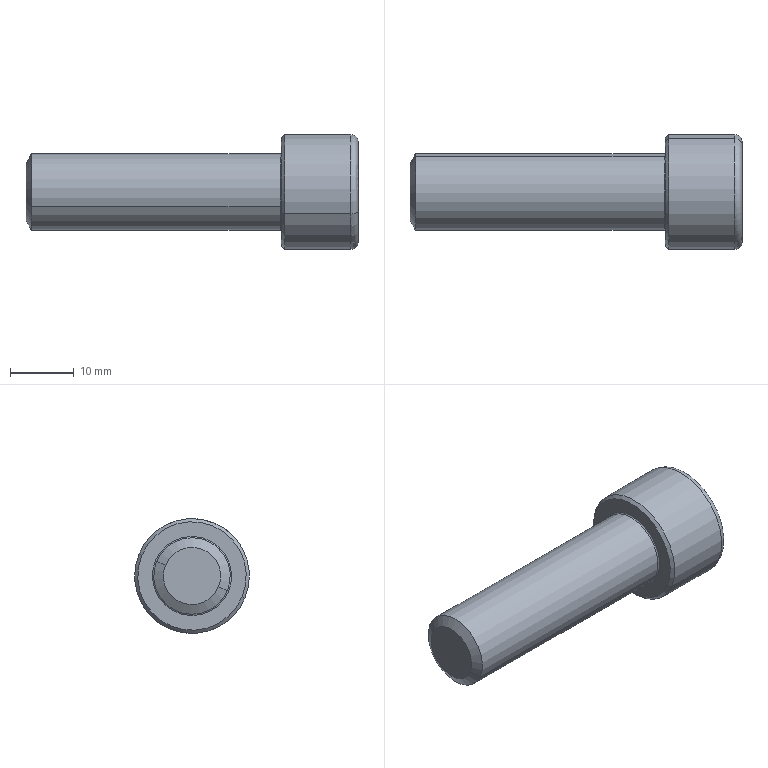Component | SolidWorks | M12_40_T70.1-1 | 1 solid | 28 faces | box 52 x 18 x 18 mm | volume 7021 mm3 | cone 10 | plane 10 | torus 4 | cylinder 4 | commonest cylinder face diameters 18 x2 12 x2 | material Plain Carbon Steel
STEP:
#1=COLOUR_RGB('',0.7922,0.8196,0.9333);
#2=FILL_AREA_STYLE_COLOUR('',#1);
#3=FILL_AREA_STYLE('',(#2));
#4=SURFACE_STYLE_FILL_AREA(#3);
#5=SURFACE_SIDE_STYLE('',(#4));
#6=SURFACE_STYLE_USAGE(.BOTH.,#5);
#7=PRESENTATION_STYLE_ASSIGNMENT((#6));
#8=CARTESIAN_POINT('',(0.122,0.3093,-1.967));
#9=VERTEX_POINT('',#8);
#10=CARTESIAN_POINT('',(0.122,-0.3093,-2.222));
#11=VERTEX_POINT('',#10);
#12=CARTESIAN_POINT('',(0.122,0.,-2.094));
#13=DIRECTION('',(-1.,0.,0.));
#14=DIRECTION('',(0.,-0.9242,-0.3818));
#15=AXIS2_PLACEMENT_3D('',#12,#13,#14);
#16=CIRCLE('',#15,0.3346);
#17=EDGE_CURVE('',#9,#11,#16,.T.);
#18=ORIENTED_EDGE('',*,*,#17,.F.);
#19=CARTESIAN_POINT('',(0.1417,0.3275,-1.959));
#20=VERTEX_POINT('',#19);
#21=CARTESIAN_POINT('',(0.1417,0.3275,-1.959));
#22=DIRECTION('',(0.7071,0.6535,0.27));
#23=VECTOR('',#22,39.37);
#24=LINE('',#21,#23);
#25=EDGE_CURVE('',#9,#20,#24,.T.);
#26=ORIENTED_EDGE('',*,*,#25,.T.);
#27=CARTESIAN_POINT('',(0.1417,-0.3275,-2.23));
#28=VERTEX_POINT('',#27);
#29=CARTESIAN_POINT('',(0.1417,0.,-2.094));
#30=DIRECTION('',(1.,0.,0.));
#31=DIRECTION('',(0.,-0.9242,-0.3818));
#32=AXIS2_PLACEMENT_3D('',#29,#30,#31);
#33=CIRCLE('',#32,0.3543);
#34=EDGE_CURVE('',#28,#20,#33,.T.);
#35=ORIENTED_EDGE('',*,*,#34,.F.);
#36=CARTESIAN_POINT('',(0.1417,-0.3275,-2.23));
#37=DIRECTION('',(0.7071,-0.6535,-0.27));
#38=VECTOR('',#37,39.37);
#39=LINE('',#36,#38);
#40=EDGE_CURVE('',#11,#28,#39,.T.);
#41=ORIENTED_EDGE('',*,*,#40,.F.);
#42=EDGE_LOOP('',(#18,#26,#35,#41));
#43=FACE_OUTER_BOUND('',#42,.T.);
#44=CARTESIAN_POINT('',(0.1417,0.,-2.094));
#45=DIRECTION('',(1.,0.,0.));
#46=DIRECTION('',(0.,-0.9242,-0.3818));
#47=AXIS2_PLACEMENT_3D('',#44,#45,#46);
#48=CONICAL_SURFACE('',#47,0.3543,0.7854);
#49=ADVANCED_FACE('',(#43),#48,.T.);
#50=CARTESIAN_POINT('',(0.5945,-0.2875,-2.213));
#51=VERTEX_POINT('',#50);
#52=CARTESIAN_POINT('',(0.5945,0.2875,-1.976));
#53=VERTEX_POINT('',#52);
#54=CARTESIAN_POINT('',(0.5945,0.,-2.094));
#55=DIRECTION('',(1.,0.,0.));
#56=DIRECTION('',(0.,0.9242,0.3818));
#57=AXIS2_PLACEMENT_3D('',#54,#55,#56);
#58=CIRCLE('',#57,0.311);
#59=EDGE_CURVE('',#51,#53,#58,.T.);
#60=ORIENTED_EDGE('',*,*,#59,.F.);
#61=CARTESIAN_POINT('',(0.5512,-0.3275,-2.23));
#62=VERTEX_POINT('',#61);
#63=CARTESIAN_POINT('',(0.5512,-0.2875,-2.213));
#64=DIRECTION('',(0.,0.3818,-0.9242));
#65=DIRECTION('',(0.,0.9242,0.3818));
#66=AXIS2_PLACEMENT_3D('',#63,#64,#65);
#67=CIRCLE('',#66,0.04331);
#68=EDGE_CURVE('',#51,#62,#67,.T.);
#69=ORIENTED_EDGE('',*,*,#68,.T.);
#70=CARTESIAN_POINT('',(0.5512,0.3275,-1.959));
#71=VERTEX_POINT('',#70);
#72=CARTESIAN_POINT('',(0.5512,0.,-2.094));
#73=DIRECTION('',(-1.,0.,0.));
#74=DIRECTION('',(0.,0.9242,0.3818));
#75=AXIS2_PLACEMENT_3D('',#72,#73,#74);
#76=CIRCLE('',#75,0.3543);
#77=EDGE_CURVE('',#71,#62,#76,.T.);
#78=ORIENTED_EDGE('',*,*,#77,.F.);
#79=CARTESIAN_POINT('',(0.5512,0.2875,-1.976));
#80=DIRECTION('',(0.,-0.3818,0.9242));
#81=DIRECTION('',(0.,-0.9242,-0.3818));
#82=AXIS2_PLACEMENT_3D('',#79,#80,#81);
#83=CIRCLE('',#82,0.04331);
#84=EDGE_CURVE('',#53,#71,#83,.T.);
#85=ORIENTED_EDGE('',*,*,#84,.F.);
#86=EDGE_LOOP('',(#60,#69,#78,#85));
#87=FACE_OUTER_BOUND('',#86,.T.);
#88=CARTESIAN_POINT('',(0.5512,0.,-2.094));
#89=DIRECTION('',(-1.,0.,0.));
#90=DIRECTION('',(0.,0.9242,0.3818));
#91=AXIS2_PLACEMENT_3D('',#88,#89,#90);
#92=TOROIDAL_SURFACE('',#91,0.311,0.04331);
#93=ADVANCED_FACE('',(#87),#92,.T.);
#94=CARTESIAN_POINT('',(-1.453,-0.1632,-2.162));
#95=VERTEX_POINT('',#94);
#96=CARTESIAN_POINT('',(-1.453,0.1632,-2.027));
#97=VERTEX_POINT('',#96);
#98=CARTESIAN_POINT('',(-1.453,0.,-2.094));
#99=DIRECTION('',(1.,0.,0.));
#100=DIRECTION('',(0.,-0.9242,-0.3818));
#101=AXIS2_PLACEMENT_3D('',#98,#99,#100);
#102=CIRCLE('',#101,0.1766);
#103=EDGE_CURVE('',#95,#97,#102,.T.);
#104=ORIENTED_EDGE('',*,*,#103,.T.);
#105=CARTESIAN_POINT('',(-1.418,0.2183,-2.004));
#106=VERTEX_POINT('',#105);
#107=CARTESIAN_POINT('',(-1.418,0.2183,-2.004));
#108=DIRECTION('',(0.5,0.8004,0.3307));
#109=VECTOR('',#108,39.37);
#110=LINE('',#107,#109);
#111=EDGE_CURVE('',#97,#106,#110,.T.);
#112=ORIENTED_EDGE('',*,*,#111,.T.);
#113=CARTESIAN_POINT('',(-1.418,-0.2183,-2.185));
#114=VERTEX_POINT('',#113);
#115=CARTESIAN_POINT('',(-1.418,0.,-2.094));
#116=DIRECTION('',(1.,0.,0.));
#117=DIRECTION('',(0.,-0.9242,-0.3818));
#118=AXIS2_PLACEMENT_3D('',#115,#116,#117);
#119=CIRCLE('',#118,0.2362);
#120=EDGE_CURVE('',#114,#106,#119,.T.);
#121=ORIENTED_EDGE('',*,*,#120,.F.);
#122=CARTESIAN_POINT('',(-1.418,-0.2183,-2.185));
#123=DIRECTION('',(0.5,-0.8004,-0.3307));
#124=VECTOR('',#123,39.37);
#125=LINE('',#122,#124);
#126=EDGE_CURVE('',#95,#114,#125,.T.);
#127=ORIENTED_EDGE('',*,*,#126,.F.);
#128=EDGE_LOOP('',(#104,#112,#121,#127));
#129=FACE_OUTER_BOUND('',#128,.T.);
#130=CARTESIAN_POINT('',(-1.418,0.,-2.094));
#131=DIRECTION('',(1.,0.,0.));
#132=DIRECTION('',(0.,-0.9242,-0.3818));
#133=AXIS2_PLACEMENT_3D('',#130,#131,#132);
#134=CONICAL_SURFACE('',#133,0.2362,1.047);
#135=ADVANCED_FACE('',(#129),#134,.T.);
#136=CARTESIAN_POINT('',(0.122,0.2256,-2.001));
#137=VERTEX_POINT('',#136);
#138=CARTESIAN_POINT('',(0.122,-0.2256,-2.188));
#139=VERTEX_POINT('',#138);
#140=CARTESIAN_POINT('',(0.122,0.,-2.094));
#141=DIRECTION('',(1.,0.,0.));
#142=DIRECTION('',(0.,-0.9242,-0.3818));
#143=AXIS2_PLACEMENT_3D('',#140,#141,#142);
#144=CIRCLE('',#143,0.2441);
#145=EDGE_CURVE('',#137,#139,#144,.T.);
#146=ORIENTED_EDGE('',*,*,#145,.F.);
#147=CARTESIAN_POINT('',(0.1142,0.2183,-2.004));
#148=VERTEX_POINT('',#147);
#149=CARTESIAN_POINT('',(0.1142,0.2256,-2.001));
#150=DIRECTION('',(0.,0.3818,-0.9242));
#151=DIRECTION('',(0.,0.9242,0.3818));
#152=AXIS2_PLACEMENT_3D('',#149,#150,#151);
#153=CIRCLE('',#152,0.007874);
#154=EDGE_CURVE('',#137,#148,#153,.T.);
#155=ORIENTED_EDGE('',*,*,#154,.T.);
#156=CARTESIAN_POINT('',(0.1142,-0.2183,-2.185));
#157=VERTEX_POINT('',#156);
#158=CARTESIAN_POINT('',(0.1142,0.,-2.094));
#159=DIRECTION('',(1.,0.,0.));
#160=DIRECTION('',(0.,-0.9242,-0.3818));
#161=AXIS2_PLACEMENT_3D('',#158,#159,#160);
#162=CIRCLE('',#161,0.2362);
#163=EDGE_CURVE('',#148,#157,#162,.T.);
#164=ORIENTED_EDGE('',*,*,#163,.T.);
#165=CARTESIAN_POINT('',(0.1142,-0.2256,-2.188));
#166=DIRECTION('',(0.,-0.3818,0.9242));
#167=DIRECTION('',(0.,-0.9242,-0.3818));
#168=AXIS2_PLACEMENT_3D('',#165,#166,#167);
#169=CIRCLE('',#168,0.007874);
#170=EDGE_CURVE('',#139,#157,#169,.T.);
#171=ORIENTED_EDGE('',*,*,#170,.F.);
#172=EDGE_LOOP('',(#146,#155,#164,#171));
#173=FACE_OUTER_BOUND('',#172,.T.);
#174=CARTESIAN_POINT('',(0.1142,0.,-2.094));
#175=DIRECTION('',(1.,0.,0.));
#176=DIRECTION('',(0.,-0.9242,-0.3818));
#177=AXIS2_PLACEMENT_3D('',#174,#175,#176);
#178=TOROIDAL_SURFACE('',#177,0.2441,0.007874);
#179=ADVANCED_FACE('',(#173),#178,.F.);
#180=ORIENTED_EDGE('',*,*,#34,.T.);
#181=CARTESIAN_POINT('',(0.5945,0.3275,-1.959));
#182=DIRECTION('',(1.,0.,0.));
#183=VECTOR('',#182,39.37);
#184=LINE('',#181,#183);
#185=EDGE_CURVE('',#20,#71,#184,.T.);
#186=ORIENTED_EDGE('',*,*,#185,.T.);
#187=ORIENTED_EDGE('',*,*,#77,.T.);
#188=CARTESIAN_POINT('',(0.5945,-0.3275,-2.23));
#189=DIRECTION('',(1.,0.,0.));
#190=VECTOR('',#189,39.37);
#191=LINE('',#188,#190);
#192=EDGE_CURVE('',#28,#62,#191,.T.);
#193=ORIENTED_EDGE('',*,*,#192,.F.);
#194=EDGE_LOOP('',(#180,#186,#187,#193));
#195=FACE_OUTER_BOUND('',#194,.T.);
#196=CARTESIAN_POINT('',(0.5945,0.,-2.094));
#197=DIRECTION('',(1.,0.,0.));
#198=DIRECTION('',(0.,-0.9242,-0.3818));
#199=AXIS2_PLACEMENT_3D('',#196,#197,#198);
#200=CYLINDRICAL_SURFACE('',#199,0.3543);
#201=ADVANCED_FACE('',(#195),#200,.T.);
#202=ORIENTED_EDGE('',*,*,#120,.T.);
#203=CARTESIAN_POINT('',(0.5945,0.2183,-2.004));
#204=DIRECTION('',(1.,0.,0.));
#205=VECTOR('',#204,39.37);
#206=LINE('',#203,#205);
#207=EDGE_CURVE('',#106,#148,#206,.T.);
#208=ORIENTED_EDGE('',*,*,#207,.T.);
#209=CARTESIAN_POINT('',(0.1142,0.,-2.094));
#210=DIRECTION('',(1.,0.,0.));
#211=DIRECTION('',(0.,-0.9242,-0.3818));
#212=AXIS2_PLACEMENT_3D('',#209,#210,#211);
#213=CIRCLE('',#212,0.2362);
#214=EDGE_CURVE('',#157,#148,#213,.T.);
#215=ORIENTED_EDGE('',*,*,#214,.F.);
#216=CARTESIAN_POINT('',(0.5945,-0.2183,-2.185));
#217=DIRECTION('',(1.,0.,0.));
#218=VECTOR('',#217,39.37);
#219=LINE('',#216,#218);
#220=EDGE_CURVE('',#114,#157,#219,.T.);
#221=ORIENTED_EDGE('',*,*,#220,.F.);
#222=EDGE_LOOP('',(#202,#208,#215,#221));
#223=FACE_OUTER_BOUND('',#222,.T.);
#224=CARTESIAN_POINT('',(0.5945,0.,-2.094));
#225=DIRECTION('',(1.,0.,0.));
#226=DIRECTION('',(0.,-0.9242,-0.3818));
#227=AXIS2_PLACEMENT_3D('',#224,#225,#226);
#228=CYLINDRICAL_SURFACE('',#227,0.2362);
#229=ADVANCED_FACE('',(#223),#228,.T.);
#230=ORIENTED_EDGE('',*,*,#207,.F.);
#231=CARTESIAN_POINT('',(-1.418,0.,-2.094));
#232=DIRECTION('',(1.,0.,0.));
#233=DIRECTION('',(0.,-0.9242,-0.3818));
#234=AXIS2_PLACEMENT_3D('',#231,#232,#233);
#235=CIRCLE('',#234,0.2362);
#236=EDGE_CURVE('',#106,#114,#235,.T.);
#237=ORIENTED_EDGE('',*,*,#236,.T.);
#238=ORIENTED_EDGE('',*,*,#220,.T.);
#239=ORIENTED_EDGE('',*,*,#163,.F.);
#240=EDGE_LOOP('',(#230,#237,#238,#239));
#241=FACE_OUTER_BOUND('',#240,.T.);
#242=CARTESIAN_POINT('',(0.5945,0.,-2.094));
#243=DIRECTION('',(1.,0.,0.));
#244=DIRECTION('',(0.,-0.9242,-0.3818));
#245=AXIS2_PLACEMENT_3D('',#242,#243,#244);
#246=CYLINDRICAL_SURFACE('',#245,0.2362);
#247=ADVANCED_FACE('',(#241),#246,.T.);
#248=CARTESIAN_POINT('',(0.5945,0.,-2.094));
#249=DIRECTION('',(1.,0.,0.));
#250=DIRECTION('',(0.,0.9242,0.3818));
#251=AXIS2_PLACEMENT_3D('',#248,#249,#250);
#252=CIRCLE('',#251,0.311);
#253=EDGE_CURVE('',#53,#51,#252,.T.);
#254=ORIENTED_EDGE('',*,*,#253,.T.);
#255=ORIENTED_EDGE('',*,*,#59,.T.);
#256=EDGE_LOOP('',(#254,#255));
#257=FACE_OUTER_BOUND('',#256,.T.);
#258=CARTESIAN_POINT('',(0.5945,0.208,-2.009));
#259=VERTEX_POINT('',#258);
#260=CARTESIAN_POINT('',(0.5945,0.02957,-1.871));
#261=VERTEX_POINT('',#260);
#262=CARTESIAN_POINT('',(0.5945,0.,-2.094));
#263=DIRECTION('',(1.,0.,0.));
#264=DIRECTION('',(0.,-0.9242,-0.3818));
#265=AXIS2_PLACEMENT_3D('',#262,#263,#264);
#266=CIRCLE('',#265,0.225);
#267=EDGE_CURVE('',#259,#261,#266,.T.);
#268=ORIENTED_EDGE('',*,*,#267,.F.);
#269=CARTESIAN_POINT('',(0.5945,0.1784,-2.232));
#270=VERTEX_POINT('',#269);
#271=CARTESIAN_POINT('',(0.5945,0.,-2.094));
#272=DIRECTION('',(1.,0.,0.));
#273=DIRECTION('',(0.,-0.9242,-0.3818));
#274=AXIS2_PLACEMENT_3D('',#271,#272,#273);
#275=CIRCLE('',#274,0.225);
#276=EDGE_CURVE('',#270,#259,#275,.T.);
#277=ORIENTED_EDGE('',*,*,#276,.F.);
#278=CARTESIAN_POINT('',(0.5945,-0.02957,-2.318));
#279=VERTEX_POINT('',#278);
#280=CARTESIAN_POINT('',(0.5945,0.,-2.094));
#281=DIRECTION('',(1.,0.,0.));
#282=DIRECTION('',(0.,-0.9242,-0.3818));
#283=AXIS2_PLACEMENT_3D('',#280,#281,#282);
#284=CIRCLE('',#283,0.225);
#285=EDGE_CURVE('',#279,#270,#284,.T.);
#286=ORIENTED_EDGE('',*,*,#285,.F.);
#287=CARTESIAN_POINT('',(0.5945,-0.208,-2.18));
#288=VERTEX_POINT('',#287);
#289=CARTESIAN_POINT('',(0.5945,0.,-2.094));
#290=DIRECTION('',(1.,0.,0.));
#291=DIRECTION('',(0.,-0.9242,-0.3818));
#292=AXIS2_PLACEMENT_3D('',#289,#290,#291);
#293=CIRCLE('',#292,0.225);
#294=EDGE_CURVE('',#288,#279,#293,.T.);
#295=ORIENTED_EDGE('',*,*,#294,.F.);
#296=CARTESIAN_POINT('',(0.5945,-0.1784,-1.957));
#297=VERTEX_POINT('',#296);
#298=CARTESIAN_POINT('',(0.5945,0.,-2.094));
#299=DIRECTION('',(1.,0.,0.));
#300=DIRECTION('',(0.,-0.9242,-0.3818));
#301=AXIS2_PLACEMENT_3D('',#298,#299,#300);
#302=CIRCLE('',#301,0.225);
#303=EDGE_CURVE('',#297,#288,#302,.T.);
#304=ORIENTED_EDGE('',*,*,#303,.F.);
#305=CARTESIAN_POINT('',(0.5945,0.,-2.094));
#306=DIRECTION('',(1.,0.,0.));
#307=DIRECTION('',(0.,-0.9242,-0.3818));
#308=AXIS2_PLACEMENT_3D('',#305,#306,#307);
#309=CIRCLE('',#308,0.225);
#310=EDGE_CURVE('',#261,#297,#309,.T.);
#311=ORIENTED_EDGE('',*,*,#310,.F.);
#312=EDGE_LOOP('',(#268,#277,#286,#295,#304,#311));
#313=FACE_BOUND('',#312,.T.);
#314=CARTESIAN_POINT('',(0.5945,0.,-2.094));
#315=DIRECTION('',(-1.,0.,0.));
#316=DIRECTION('',(0.,0.9242,0.3818));
#317=AXIS2_PLACEMENT_3D('',#314,#315,#316);
#318=PLANE('',#317);
#319=ADVANCED_FACE('',(#257,#313),#318,.F.);
#320=ORIENTED_EDGE('',*,*,#185,.F.);
#321=CARTESIAN_POINT('',(0.1417,0.,-2.094));
#322=DIRECTION('',(1.,0.,0.));
#323=DIRECTION('',(0.,-0.9242,-0.3818));
#324=AXIS2_PLACEMENT_3D('',#321,#322,#323);
#325=CIRCLE('',#324,0.3543);
#326=EDGE_CURVE('',#20,#28,#325,.T.);
#327=ORIENTED_EDGE('',*,*,#326,.T.);
#328=ORIENTED_EDGE('',*,*,#192,.T.);
#329=CARTESIAN_POINT('',(0.5512,0.,-2.094));
#330=DIRECTION('',(-1.,0.,0.));
#331=DIRECTION('',(0.,0.9242,0.3818));
#332=AXIS2_PLACEMENT_3D('',#329,#330,#331);
#333=CIRCLE('',#332,0.3543);
#334=EDGE_CURVE('',#62,#71,#333,.T.);
#335=ORIENTED_EDGE('',*,*,#334,.T.);
#336=EDGE_LOOP('',(#320,#327,#328,#335));
#337=FACE_OUTER_BOUND('',#336,.T.);
#338=CARTESIAN_POINT('',(0.5945,0.,-2.094));
#339=DIRECTION('',(1.,0.,0.));
#340=DIRECTION('',(0.,-0.9242,-0.3818));
#341=AXIS2_PLACEMENT_3D('',#338,#339,#340);
#342=CYLINDRICAL_SURFACE('',#341,0.3543);
#343=ADVANCED_FACE('',(#337),#342,.T.);
#344=CARTESIAN_POINT('',(0.122,0.,-2.094));
#345=DIRECTION('',(-1.,0.,0.));
#346=DIRECTION('',(0.,-0.9242,-0.3818));
#347=AXIS2_PLACEMENT_3D('',#344,#345,#346);
#348=CIRCLE('',#347,0.3346);
#349=EDGE_CURVE('',#11,#9,#348,.T.);
#350=ORIENTED_EDGE('',*,*,#349,.T.);
#351=ORIENTED_EDGE('',*,*,#17,.T.);
#352=EDGE_LOOP('',(#350,#351));
#353=FACE_OUTER_BOUND('',#352,.T.);
#354=CARTESIAN_POINT('',(0.122,0.,-2.094));
#355=DIRECTION('',(1.,0.,0.));
#356=DIRECTION('',(0.,-0.9242,-0.3818));
#357=AXIS2_PLACEMENT_3D('',#354,#355,#356);
#358=CIRCLE('',#357,0.2441);
#359=EDGE_CURVE('',#139,#137,#358,.T.);
#360=ORIENTED_EDGE('',*,*,#359,.T.);
#361=ORIENTED_EDGE('',*,*,#145,.T.);
#362=EDGE_LOOP('',(#360,#361));
#363=FACE_BOUND('',#362,.T.);
#364=CARTESIAN_POINT('',(0.122,0.1353,-2.422));
#365=DIRECTION('',(1.,0.,0.));
#366=DIRECTION('',(0.,-0.9242,-0.3818));
#367=AXIS2_PLACEMENT_3D('',#364,#365,#366);
#368=PLANE('',#367);
#369=ADVANCED_FACE('',(#353,#363),#368,.F.);
#370=ORIENTED_EDGE('',*,*,#154,.F.);
#371=ORIENTED_EDGE('',*,*,#359,.F.);
#372=ORIENTED_EDGE('',*,*,#170,.T.);
#373=ORIENTED_EDGE('',*,*,#214,.T.);
#374=EDGE_LOOP('',(#370,#371,#372,#373));
#375=FACE_OUTER_BOUND('',#374,.T.);
#376=CARTESIAN_POINT('',(0.1142,0.,-2.094));
#377=DIRECTION('',(1.,0.,0.));
#378=DIRECTION('',(0.,-0.9242,-0.3818));
#379=AXIS2_PLACEMENT_3D('',#376,#377,#378);
#380=TOROIDAL_SURFACE('',#379,0.2441,0.007874);
#381=ADVANCED_FACE('',(#375),#380,.F.);
#382=ORIENTED_EDGE('',*,*,#111,.F.);
#383=CARTESIAN_POINT('',(-1.453,0.,-2.094));
#384=DIRECTION('',(1.,0.,0.));
#385=DIRECTION('',(0.,-0.9242,-0.3818));
#386=AXIS2_PLACEMENT_3D('',#383,#384,#385);
#387=CIRCLE('',#386,0.1766);
#388=EDGE_CURVE('',#97,#95,#387,.T.);
#389=ORIENTED_EDGE('',*,*,#388,.T.);
#390=ORIENTED_EDGE('',*,*,#126,.T.);
#391=ORIENTED_EDGE('',*,*,#236,.F.);
#392=EDGE_LOOP('',(#382,#389,#390,#391));
#393=FACE_OUTER_BOUND('',#392,.T.);
#394=CARTESIAN_POINT('',(-1.418,0.,-2.094));
#395=DIRECTION('',(1.,0.,0.));
#396=DIRECTION('',(0.,-0.9242,-0.3818));
#397=AXIS2_PLACEMENT_3D('',#394,#395,#396);
#398=CONICAL_SURFACE('',#397,0.2362,1.047);
#399=ADVANCED_FACE('',(#393),#398,.T.);
#400=ORIENTED_EDGE('',*,*,#103,.F.);
#401=ORIENTED_EDGE('',*,*,#388,.F.);
#402=EDGE_LOOP('',(#400,#401));
#403=FACE_OUTER_BOUND('',#402,.T.);
#404=CARTESIAN_POINT('',(-1.453,0.0902,-2.313));
#405=DIRECTION('',(1.,0.,0.));
#406=DIRECTION('',(0.,-0.9242,-0.3818));
#407=AXIS2_PLACEMENT_3D('',#404,#405,#406);
#408=PLANE('',#407);
#409=ADVANCED_FACE('',(#403),#408,.F.);
#410=ORIENTED_EDGE('',*,*,#68,.F.);
#411=ORIENTED_EDGE('',*,*,#253,.F.);
#412=ORIENTED_EDGE('',*,*,#84,.T.);
#413=ORIENTED_EDGE('',*,*,#334,.F.);
#414=EDGE_LOOP('',(#410,#411,#412,#413));
#415=FACE_OUTER_BOUND('',#414,.T.);
#416=CARTESIAN_POINT('',(0.5512,0.,-2.094));
#417=DIRECTION('',(-1.,0.,0.));
#418=DIRECTION('',(0.,0.9242,0.3818));
#419=AXIS2_PLACEMENT_3D('',#416,#417,#418);
#420=TOROIDAL_SURFACE('',#419,0.311,0.04331);
#421=ADVANCED_FACE('',(#415),#420,.T.);
#422=ORIENTED_EDGE('',*,*,#25,.F.);
#423=ORIENTED_EDGE('',*,*,#349,.F.);
#424=ORIENTED_EDGE('',*,*,#40,.T.);
#425=ORIENTED_EDGE('',*,*,#326,.F.);
#426=EDGE_LOOP('',(#422,#423,#424,#425));
#427=FACE_OUTER_BOUND('',#426,.T.);
#428=CARTESIAN_POINT('',(0.1417,0.,-2.094));
#429=DIRECTION('',(1.,0.,0.));
#430=DIRECTION('',(0.,-0.9242,-0.3818));
#431=AXIS2_PLACEMENT_3D('',#428,#429,#430);
#432=CONICAL_SURFACE('',#431,0.3543,0.7854);
#433=ADVANCED_FACE('',(#427),#432,.T.);
#434=ORIENTED_EDGE('',*,*,#294,.T.);
#435=CARTESIAN_POINT('',(0.5945,-0.208,-2.18));
#436=CARTESIAN_POINT('',(0.5839,-0.1788,-2.203));
#437=CARTESIAN_POINT('',(0.5771,-0.1493,-2.226));
#438=CARTESIAN_POINT('',(0.5771,-0.1113,-2.255));
#439=CARTESIAN_POINT('',(0.5775,-0.1037,-2.261));
#440=CARTESIAN_POINT('',(0.5791,-0.08866,-2.272));
#441=CARTESIAN_POINT('',(0.5802,-0.08117,-2.278));
#442=CARTESIAN_POINT('',(0.5848,-0.05885,-2.295));
#443=CARTESIAN_POINT('',(0.5892,-0.04415,-2.306));
#444=CARTESIAN_POINT('',(0.5945,-0.02957,-2.318));
#445=B_SPLINE_CURVE_WITH_KNOTS('',3,(#435,#436,#437,#438,#439,#440,#441,#442,#443,#444),.UNSPECIFIED.,.F.,.F.,(4,2,2,2,4),(0.00000024,0.002886,0.003608,0.004329,0.005772),.UNSPECIFIED.);
#446=EDGE_CURVE('',#288,#279,#445,.T.);
#447=ORIENTED_EDGE('',*,*,#446,.F.);
#448=EDGE_LOOP('',(#434,#447));
#449=FACE_OUTER_BOUND('',#448,.T.);
#450=CARTESIAN_POINT('',(0.5945,0.,-2.094));
#451=DIRECTION('',(1.,0.,0.));
#452=DIRECTION('',(0.,-0.9242,-0.3818));
#453=AXIS2_PLACEMENT_3D('',#450,#451,#452);
#454=CONICAL_SURFACE('',#453,0.225,1.047);
#455=ADVANCED_FACE('',(#449),#454,.F.);
#456=ORIENTED_EDGE('',*,*,#285,.T.);
#457=CARTESIAN_POINT('',(0.5945,-0.02957,-2.318));
#458=CARTESIAN_POINT('',(0.5892,-0.01276,-2.311));
#459=CARTESIAN_POINT('',(0.5849,0.00427,-2.304));
#460=CARTESIAN_POINT('',(0.5788,0.03903,-2.289));
#461=CARTESIAN_POINT('',(0.5771,0.05682,-2.282));
#462=CARTESIAN_POINT('',(0.5771,0.09194,-2.267));
#463=CARTESIAN_POINT('',(0.5787,0.1094,-2.26));
#464=CARTESIAN_POINT('',(0.5848,0.1442,-2.246));
#465=CARTESIAN_POINT('',(0.5892,0.1615,-2.239));
#466=CARTESIAN_POINT('',(0.5945,0.1784,-2.232));
#467=B_SPLINE_CURVE_WITH_KNOTS('',3,(#457,#458,#459,#460,#461,#462,#463,#464,#465,#466),.UNSPECIFIED.,.F.,.F.,(4,2,2,2,4),(0.0153,0.01675,0.0182,0.01964,0.02109),.UNSPECIFIED.);
#468=EDGE_CURVE('',#279,#270,#467,.T.);
#469=ORIENTED_EDGE('',*,*,#468,.F.);
#470=EDGE_LOOP('',(#456,#469));
#471=FACE_OUTER_BOUND('',#470,.T.);
#472=CARTESIAN_POINT('',(0.5945,0.,-2.094));
#473=DIRECTION('',(1.,0.,0.));
#474=DIRECTION('',(0.,-0.9242,-0.3818));
#475=AXIS2_PLACEMENT_3D('',#472,#473,#474);
#476=CONICAL_SURFACE('',#475,0.225,1.047);
#477=ADVANCED_FACE('',(#471),#476,.F.);
#478=ORIENTED_EDGE('',*,*,#276,.T.);
#479=CARTESIAN_POINT('',(0.5945,0.1784,-2.232));
#480=CARTESIAN_POINT('',(0.5839,0.1832,-2.195));
#481=CARTESIAN_POINT('',(0.5771,0.1881,-2.158));
#482=CARTESIAN_POINT('',(0.5771,0.1944,-2.111));
#483=CARTESIAN_POINT('',(0.5775,0.1957,-2.101));
#484=CARTESIAN_POINT('',(0.5791,0.1982,-2.082));
#485=CARTESIAN_POINT('',(0.5802,0.1994,-2.073));
#486=CARTESIAN_POINT('',(0.5848,0.2031,-2.045));
#487=CARTESIAN_POINT('',(0.5892,0.2055,-2.027));
#488=CARTESIAN_POINT('',(0.5945,0.208,-2.009));
#489=B_SPLINE_CURVE_WITH_KNOTS('',3,(#479,#480,#481,#482,#483,#484,#485,#486,#487,#488),.UNSPECIFIED.,.F.,.F.,(4,2,2,2,4),(0.00000024,0.002886,0.003608,0.004329,0.005772),.UNSPECIFIED.);
#490=EDGE_CURVE('',#270,#259,#489,.T.);
#491=ORIENTED_EDGE('',*,*,#490,.F.);
#492=EDGE_LOOP('',(#478,#491));
#493=FACE_OUTER_BOUND('',#492,.T.);
#494=CARTESIAN_POINT('',(0.5945,0.,-2.094));
#495=DIRECTION('',(1.,0.,0.));
#496=DIRECTION('',(0.,-0.9242,-0.3818));
#497=AXIS2_PLACEMENT_3D('',#494,#495,#496);
#498=CONICAL_SURFACE('',#497,0.225,1.047);
#499=ADVANCED_FACE('',(#493),#498,.F.);
#500=ORIENTED_EDGE('',*,*,#267,.T.);
#501=CARTESIAN_POINT('',(0.5945,0.208,-2.009));
#502=CARTESIAN_POINT('',(0.5839,0.1788,-1.986));
#503=CARTESIAN_POINT('',(0.5771,0.1493,-1.963));
#504=CARTESIAN_POINT('',(0.5771,0.1113,-1.934));
#505=CARTESIAN_POINT('',(0.5775,0.1037,-1.928));
#506=CARTESIAN_POINT('',(0.5791,0.08866,-1.917));
#507=CARTESIAN_POINT('',(0.5802,0.08117,-1.911));
#508=CARTESIAN_POINT('',(0.5848,0.05885,-1.894));
#509=CARTESIAN_POINT('',(0.5892,0.04415,-1.883));
#510=CARTESIAN_POINT('',(0.5945,0.02957,-1.871));
#511=B_SPLINE_CURVE_WITH_KNOTS('',3,(#501,#502,#503,#504,#505,#506,#507,#508,#509,#510),.UNSPECIFIED.,.F.,.F.,(4,2,2,2,4),(0.00000024,0.002886,0.003608,0.004329,0.005772),.UNSPECIFIED.);
#512=EDGE_CURVE('',#259,#261,#511,.T.);
#513=ORIENTED_EDGE('',*,*,#512,.F.);
#514=EDGE_LOOP('',(#500,#513));
#515=FACE_OUTER_BOUND('',#514,.T.);
#516=CARTESIAN_POINT('',(0.5945,0.,-2.094));
#517=DIRECTION('',(1.,0.,0.));
#518=DIRECTION('',(0.,-0.9242,-0.3818));
#519=AXIS2_PLACEMENT_3D('',#516,#517,#518);
#520=CONICAL_SURFACE('',#519,0.225,1.047);
#521=ADVANCED_FACE('',(#515),#520,.F.);
#522=ORIENTED_EDGE('',*,*,#310,.T.);
#523=CARTESIAN_POINT('',(0.5945,0.02957,-1.871));
#524=CARTESIAN_POINT('',(0.5892,0.01267,-1.878));
#525=CARTESIAN_POINT('',(0.5848,-0.004645,-1.886));
#526=CARTESIAN_POINT('',(0.5787,-0.03941,-1.9));
#527=CARTESIAN_POINT('',(0.5771,-0.05687,-1.907));
#528=CARTESIAN_POINT('',(0.5771,-0.09199,-1.922));
#529=CARTESIAN_POINT('',(0.5788,-0.1098,-1.929));
#530=CARTESIAN_POINT('',(0.5849,-0.1445,-1.943));
#531=CARTESIAN_POINT('',(0.5892,-0.1616,-1.95));
#532=CARTESIAN_POINT('',(0.5945,-0.1784,-1.957));
#533=B_SPLINE_CURVE_WITH_KNOTS('',3,(#523,#524,#525,#526,#527,#528,#529,#530,#531,#532),.UNSPECIFIED.,.F.,.F.,(4,2,2,2,4),(0.0049,0.006345,0.00779,0.009234,0.01068),.UNSPECIFIED.);
#534=EDGE_CURVE('',#261,#297,#533,.T.);
#535=ORIENTED_EDGE('',*,*,#534,.F.);
#536=EDGE_LOOP('',(#522,#535));
#537=FACE_OUTER_BOUND('',#536,.T.);
#538=CARTESIAN_POINT('',(0.5945,0.,-2.094));
#539=DIRECTION('',(1.,0.,0.));
#540=DIRECTION('',(0.,-0.9242,-0.3818));
#541=AXIS2_PLACEMENT_3D('',#538,#539,#540);
#542=CONICAL_SURFACE('',#541,0.225,1.047);
#543=ADVANCED_FACE('',(#537),#542,.F.);
#544=ORIENTED_EDGE('',*,*,#303,.T.);
#545=CARTESIAN_POINT('',(0.5945,-0.1784,-1.957));
#546=CARTESIAN_POINT('',(0.5839,-0.1832,-1.994));
#547=CARTESIAN_POINT('',(0.5771,-0.1881,-2.031));
#548=CARTESIAN_POINT('',(0.5771,-0.1944,-2.078));
#549=CARTESIAN_POINT('',(0.5775,-0.1957,-2.088));
#550=CARTESIAN_POINT('',(0.5791,-0.1982,-2.107));
#551=CARTESIAN_POINT('',(0.5802,-0.1994,-2.116));
#552=CARTESIAN_POINT('',(0.5848,-0.2031,-2.144));
#553=CARTESIAN_POINT('',(0.5892,-0.2055,-2.162));
#554=CARTESIAN_POINT('',(0.5945,-0.208,-2.18));
#555=B_SPLINE_CURVE_WITH_KNOTS('',3,(#545,#546,#547,#548,#549,#550,#551,#552,#553,#554),.UNSPECIFIED.,.F.,.F.,(4,2,2,2,4),(0.00000024,0.002886,0.003608,0.004329,0.005772),.UNSPECIFIED.);
#556=EDGE_CURVE('',#297,#288,#555,.T.);
#557=ORIENTED_EDGE('',*,*,#556,.F.);
#558=EDGE_LOOP('',(#544,#557));
#559=FACE_OUTER_BOUND('',#558,.T.);
#560=CARTESIAN_POINT('',(0.5945,0.,-2.094));
#561=DIRECTION('',(1.,0.,0.));
#562=DIRECTION('',(0.,-0.9242,-0.3818));
#563=AXIS2_PLACEMENT_3D('',#560,#561,#562);
#564=CONICAL_SURFACE('',#563,0.225,1.047);
#565=ADVANCED_FACE('',(#559),#564,.F.);
#566=CARTESIAN_POINT('',(0.3583,-0.1784,-1.957));
#567=VERTEX_POINT('',#566);
#568=CARTESIAN_POINT('',(0.3583,-0.208,-2.18));
#569=VERTEX_POINT('',#568);
#570=CARTESIAN_POINT('',(0.3583,-0.1784,-1.957));
#571=DIRECTION('',(0.,-0.1314,-0.9913));
#572=VECTOR('',#571,39.37);
#573=LINE('',#570,#572);
#574=EDGE_CURVE('',#567,#569,#573,.T.);
#575=ORIENTED_EDGE('',*,*,#574,.T.);
#576=CARTESIAN_POINT('',(0.3583,-0.02957,-2.318));
#577=VERTEX_POINT('',#576);
#578=CARTESIAN_POINT('',(0.3583,-0.208,-2.18));
#579=DIRECTION('',(0.,0.7928,-0.6095));
#580=VECTOR('',#579,39.37);
#581=LINE('',#578,#580);
#582=EDGE_CURVE('',#569,#577,#581,.T.);
#583=ORIENTED_EDGE('',*,*,#582,.T.);
#584=CARTESIAN_POINT('',(0.3583,0.1784,-2.232));
#585=VERTEX_POINT('',#584);
#586=CARTESIAN_POINT('',(0.3583,-0.02957,-2.318));
#587=DIRECTION('',(0.,0.9242,0.3818));
#588=VECTOR('',#587,39.37);
#589=LINE('',#586,#588);
#590=EDGE_CURVE('',#577,#585,#589,.T.);
#591=ORIENTED_EDGE('',*,*,#590,.T.);
#592=CARTESIAN_POINT('',(0.3583,0.208,-2.009));
#593=VERTEX_POINT('',#592);
#594=CARTESIAN_POINT('',(0.3583,0.1784,-2.232));
#595=DIRECTION('',(0.,0.1314,0.9913));
#596=VECTOR('',#595,39.37);
#597=LINE('',#594,#596);
#598=EDGE_CURVE('',#585,#593,#597,.T.);
#599=ORIENTED_EDGE('',*,*,#598,.T.);
#600=CARTESIAN_POINT('',(0.3583,0.02957,-1.871));
#601=VERTEX_POINT('',#600);
#602=CARTESIAN_POINT('',(0.3583,0.208,-2.009));
#603=DIRECTION('',(0.,-0.7928,0.6095));
#604=VECTOR('',#603,39.37);
#605=LINE('',#602,#604);
#606=EDGE_CURVE('',#593,#601,#605,.T.);
#607=ORIENTED_EDGE('',*,*,#606,.T.);
#608=CARTESIAN_POINT('',(0.3583,0.02957,-1.871));
#609=DIRECTION('',(0.,-0.9242,-0.3818));
#610=VECTOR('',#609,39.37);
#611=LINE('',#608,#610);
#612=EDGE_CURVE('',#601,#567,#611,.T.);
#613=ORIENTED_EDGE('',*,*,#612,.T.);
#614=EDGE_LOOP('',(#575,#583,#591,#599,#607,#613));
#615=FACE_OUTER_BOUND('',#614,.T.);
#616=CARTESIAN_POINT('',(0.3583,-0.1784,-1.957));
#617=DIRECTION('',(-1.,0.,0.));
#618=DIRECTION('',(0.,0.9242,0.3818));
#619=AXIS2_PLACEMENT_3D('',#616,#617,#618);
#620=PLANE('',#619);
#621=ADVANCED_FACE('',(#615),#620,.F.);
#622=CARTESIAN_POINT('',(0.3583,-0.208,-2.18));
#623=DIRECTION('',(1.,0.,0.));
#624=VECTOR('',#623,39.37);
#625=LINE('',#622,#624);
#626=EDGE_CURVE('',#569,#288,#625,.T.);
#627=ORIENTED_EDGE('',*,*,#626,.T.);
#628=ORIENTED_EDGE('',*,*,#446,.T.);
#629=CARTESIAN_POINT('',(0.3583,-0.02957,-2.318));
#630=DIRECTION('',(1.,0.,0.));
#631=VECTOR('',#630,39.37);
#632=LINE('',#629,#631);
#633=EDGE_CURVE('',#577,#279,#632,.T.);
#634=ORIENTED_EDGE('',*,*,#633,.F.);
#635=ORIENTED_EDGE('',*,*,#582,.F.);
#636=EDGE_LOOP('',(#627,#628,#634,#635));
#637=FACE_OUTER_BOUND('',#636,.T.);
#638=CARTESIAN_POINT('',(0.3583,-0.208,-2.18));
#639=DIRECTION('',(0.,-0.6095,-0.7928));
#640=DIRECTION('',(0.,-0.7928,0.6095));
#641=AXIS2_PLACEMENT_3D('',#638,#639,#640);
#642=PLANE('',#641);
#643=ADVANCED_FACE('',(#637),#642,.F.);
#644=ORIENTED_EDGE('',*,*,#633,.T.);
#645=ORIENTED_EDGE('',*,*,#468,.T.);
#646=CARTESIAN_POINT('',(0.3583,0.1784,-2.232));
#647=DIRECTION('',(1.,0.,0.));
#648=VECTOR('',#647,39.37);
#649=LINE('',#646,#648);
#650=EDGE_CURVE('',#585,#270,#649,.T.);
#651=ORIENTED_EDGE('',*,*,#650,.F.);
#652=ORIENTED_EDGE('',*,*,#590,.F.);
#653=EDGE_LOOP('',(#644,#645,#651,#652));
#654=FACE_OUTER_BOUND('',#653,.T.);
#655=CARTESIAN_POINT('',(0.3583,-0.02957,-2.318));
#656=DIRECTION('',(0.,0.3818,-0.9242));
#657=DIRECTION('',(0.,-0.9242,-0.3818));
#658=AXIS2_PLACEMENT_3D('',#655,#656,#657);
#659=PLANE('',#658);
#660=ADVANCED_FACE('',(#654),#659,.F.);
#661=ORIENTED_EDGE('',*,*,#650,.T.);
#662=ORIENTED_EDGE('',*,*,#490,.T.);
#663=CARTESIAN_POINT('',(0.3583,0.208,-2.009));
#664=DIRECTION('',(1.,0.,0.));
#665=VECTOR('',#664,39.37);
#666=LINE('',#663,#665);
#667=EDGE_CURVE('',#593,#259,#666,.T.);
#668=ORIENTED_EDGE('',*,*,#667,.F.);
#669=ORIENTED_EDGE('',*,*,#598,.F.);
#670=EDGE_LOOP('',(#661,#662,#668,#669));
#671=FACE_OUTER_BOUND('',#670,.T.);
#672=CARTESIAN_POINT('',(0.3583,0.1784,-2.232));
#673=DIRECTION('',(0.,0.9913,-0.1314));
#674=DIRECTION('',(0.,-0.1314,-0.9913));
#675=AXIS2_PLACEMENT_3D('',#672,#673,#674);
#676=PLANE('',#675);
#677=ADVANCED_FACE('',(#671),#676,.F.);
#678=ORIENTED_EDGE('',*,*,#667,.T.);
#679=ORIENTED_EDGE('',*,*,#512,.T.);
#680=CARTESIAN_POINT('',(0.3583,0.02957,-1.871));
#681=DIRECTION('',(1.,0.,0.));
#682=VECTOR('',#681,39.37);
#683=LINE('',#680,#682);
#684=EDGE_CURVE('',#601,#261,#683,.T.);
#685=ORIENTED_EDGE('',*,*,#684,.F.);
#686=ORIENTED_EDGE('',*,*,#606,.F.);
#687=EDGE_LOOP('',(#678,#679,#685,#686));
#688=FACE_OUTER_BOUND('',#687,.T.);
#689=CARTESIAN_POINT('',(0.3583,0.208,-2.009));
#690=DIRECTION('',(0.,0.6095,0.7928));
#691=DIRECTION('',(0.,0.7928,-0.6095));
#692=AXIS2_PLACEMENT_3D('',#689,#690,#691);
#693=PLANE('',#692);
#694=ADVANCED_FACE('',(#688),#693,.F.);
#695=ORIENTED_EDGE('',*,*,#684,.T.);
#696=ORIENTED_EDGE('',*,*,#534,.T.);
#697=CARTESIAN_POINT('',(0.3583,-0.1784,-1.957));
#698=DIRECTION('',(1.,0.,0.));
#699=VECTOR('',#698,39.37);
#700=LINE('',#697,#699);
#701=EDGE_CURVE('',#567,#297,#700,.T.);
#702=ORIENTED_EDGE('',*,*,#701,.F.);
#703=ORIENTED_EDGE('',*,*,#612,.F.);
#704=EDGE_LOOP('',(#695,#696,#702,#703));
#705=FACE_OUTER_BOUND('',#704,.T.);
#706=CARTESIAN_POINT('',(0.3583,0.02957,-1.871));
#707=DIRECTION('',(0.,-0.3818,0.9242));
#708=DIRECTION('',(0.,0.9242,0.3818));
#709=AXIS2_PLACEMENT_3D('',#706,#707,#708);
#710=PLANE('',#709);
#711=ADVANCED_FACE('',(#705),#710,.F.);
#712=ORIENTED_EDGE('',*,*,#701,.T.);
#713=ORIENTED_EDGE('',*,*,#556,.T.);
#714=ORIENTED_EDGE('',*,*,#626,.F.);
#715=ORIENTED_EDGE('',*,*,#574,.F.);
#716=EDGE_LOOP('',(#712,#713,#714,#715));
#717=FACE_OUTER_BOUND('',#716,.T.);
#718=CARTESIAN_POINT('',(0.3583,-0.1784,-1.957));
#719=DIRECTION('',(0.,-0.9913,0.1314));
#720=DIRECTION('',(0.,0.1314,0.9913));
#721=AXIS2_PLACEMENT_3D('',#718,#719,#720);
#722=PLANE('',#721);
#723=ADVANCED_FACE('',(#717),#722,.F.);
#724=CLOSED_SHELL('',(#49,#93,#135,#179,#201,#229,#247,#319,#343,#369,#381,#399,#409,#421,#433,#455,#477,#499,#521,#543,#565,#621,#643,#660,#677,#694,#711,#723));
#725=MANIFOLD_SOLID_BREP('',#724);
#726=STYLED_ITEM('',(#7),#725);
#727=(LENGTH_UNIT()NAMED_UNIT(*)SI_UNIT($,.METRE.));
#728=LENGTH_MEASURE_WITH_UNIT(LENGTH_MEASURE(0.0254),#727);
#729=DIMENSIONAL_EXPONENTS(1.,0.,0.,0.,0.,0.,0.);
#730=(CONVERSION_BASED_UNIT('',#728)LENGTH_UNIT()NAMED_UNIT(#729));
#731=UNCERTAINTY_MEASURE_WITH_UNIT(LENGTH_MEASURE(0.00001),#730,'','');
#732=(NAMED_UNIT(*)PLANE_ANGLE_UNIT()SI_UNIT($,.RADIAN.));
#733=(NAMED_UNIT(*)SI_UNIT($,.STERADIAN.)SOLID_ANGLE_UNIT());
#734=(GEOMETRIC_REPRESENTATION_CONTEXT(3)GLOBAL_UNCERTAINTY_ASSIGNED_CONTEXT((#731))GLOBAL_UNIT_ASSIGNED_CONTEXT((#730,#732,#733))REPRESENTATION_CONTEXT('',''));
#735=MECHANICAL_DESIGN_GEOMETRIC_PRESENTATION_REPRESENTATION('',(#726),#734);
#736=PRESENTATION_LAYER_ASSIGNMENT('','',(#726));
#737=CARTESIAN_POINT('',(0.,0.,0.));
#738=DIRECTION('',(0.,0.,1.));
#739=DIRECTION('',(1.,0.,0.));
#740=AXIS2_PLACEMENT_3D('',#737,#738,#739);
#741=(LENGTH_UNIT()NAMED_UNIT(*)SI_UNIT($,.METRE.));
#742=LENGTH_MEASURE_WITH_UNIT(LENGTH_MEASURE(0.0254),#741);
#743=DIMENSIONAL_EXPONENTS(1.,0.,0.,0.,0.,0.,0.);
#744=(CONVERSION_BASED_UNIT('',#742)LENGTH_UNIT()NAMED_UNIT(#743));
#745=UNCERTAINTY_MEASURE_WITH_UNIT(LENGTH_MEASURE(0.00001),#744,'','');
#746=(NAMED_UNIT(*)PLANE_ANGLE_UNIT()SI_UNIT($,.RADIAN.));
#747=(NAMED_UNIT(*)SI_UNIT($,.STERADIAN.)SOLID_ANGLE_UNIT());
#748=(GEOMETRIC_REPRESENTATION_CONTEXT(3)GLOBAL_UNCERTAINTY_ASSIGNED_CONTEXT((#745))GLOBAL_UNIT_ASSIGNED_CONTEXT((#744,#746,#747))REPRESENTATION_CONTEXT('',''));
#749=ADVANCED_BREP_SHAPE_REPRESENTATION('',(#725,#740),#748);